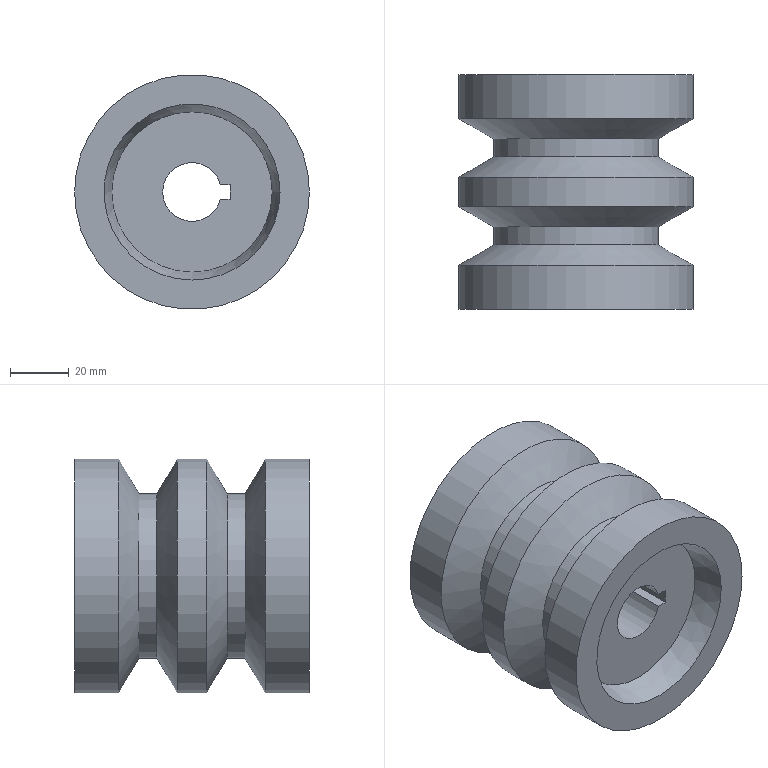Component | NX | DRIVE_WHEEL | 1 solid | 19 faces | volume 261585 mm3 | plane 7 | cone 6 | cylinder 6 | commonest cylinder face diameters 80 x3 56 x2 20 x1